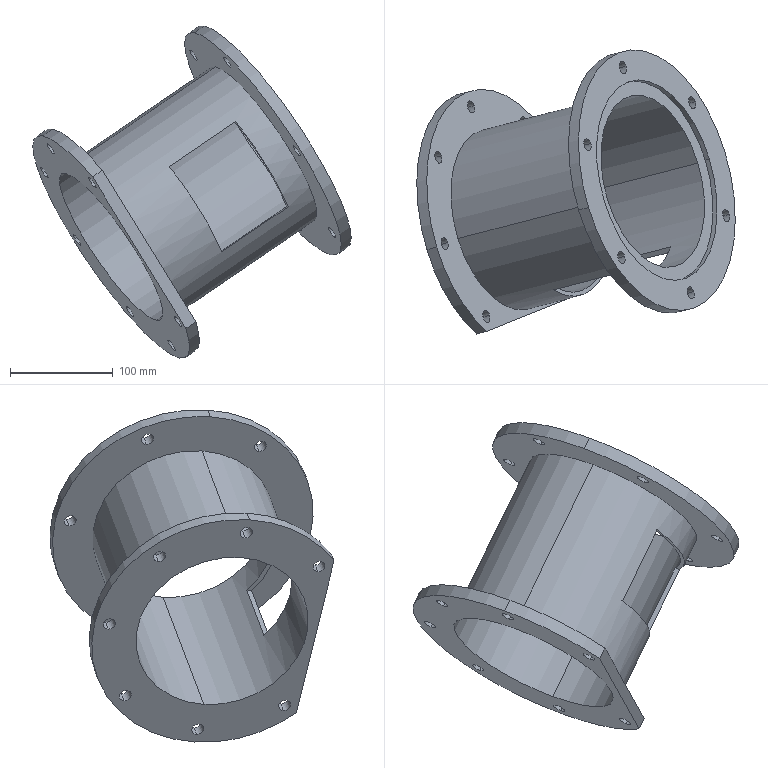Component | SolidWorks | CrusherMotorMount-1 | 1 solid | 47 faces | box 310.61 x 277.08 x 324.38 mm | volume 950992 mm3 | cylinder 37 | plane 10 | commonest cylinder face diameters 12 x26 260 x5 200 x2 180 x2 172 x2
build123d program:
from build123d import *

# Parameters (mm, degrees)
SKETCH2_R          = 6
CUT_EXTRUDE1_DEPTH = 20
CIRPATTERN1_COUNT  = 6
SKETCH3_R          = 100
CUT_EXTRUDE2_DEPTH = 5
CUT_EXTRUDE3_START = -15
SKETCH4_R          = 6
CUT_EXTRUDE3_DEPTH = 15
CIRPATTERN2_COUNT  = 8
SKETCH6_W          = 254.472
SKETCH6_H          = 74.742
CUT_EXTRUDE4_DEPTH = 20
SKETCH7_W          = 80
SKETCH7_H          = 100
CUT_EXTRUDE5_DEPTH = 269.002


with BuildPart() as part:
    # Sketch1 → Revolve1 (revolve)
    with BuildSketch(Plane.XY, mode=Mode.PRIVATE) as revolve1_sk:
        Polygon((0, 86), (0, 130), (12, 130), (12, 90), (183, 90), (183, 130), (195, 130), (195, 86), align=None)
    revolve(revolve1_sk.sketch.rotate(Axis((0, 0, 0), (1, 0, 0)), 90), axis=Axis((0, 0, 0), (1, 0, 0)))

    # Sketch2 → Cut-Extrude1 (cut)
    with BuildSketch(Plane.ZY):
        with Locations((0, 115)):
            Circle(SKETCH2_R)
    cut_extrude1 = extrude(amount=-CUT_EXTRUDE1_DEPTH, mode=Mode.SUBTRACT)

    # CirPattern1: Cut-Extrude1 ×6 about axis
    cirpattern1_axis = Axis((0, 0, 0), (1, 0, 0))
    for i in range(1, CIRPATTERN1_COUNT):
        add(cut_extrude1.rotate(cirpattern1_axis, i * 360 / CIRPATTERN1_COUNT), mode=Mode.SUBTRACT)

    # Sketch3 → Cut-Extrude2 (cut)
    with BuildSketch(Plane.ZY):
        Circle(SKETCH3_R)
    extrude(amount=-CUT_EXTRUDE2_DEPTH, mode=Mode.SUBTRACT)

    # Sketch4 → Cut-Extrude3 (cut)
    with BuildSketch(Plane(origin=(195, 0, 0), x_dir=(0, 0, -1), z_dir=(1, 0, 0)).offset(CUT_EXTRUDE3_START)):
        with Locations(Location((0, 115, 0), (0, 0, 180))):
            Circle(SKETCH4_R)
    cut_extrude3 = extrude(amount=CUT_EXTRUDE3_DEPTH, mode=Mode.SUBTRACT)

    # CirPattern2: Cut-Extrude3 ×8 about axis
    cirpattern2_axis = Axis((0, 0, 0), (1, 0, 0))
    for i in range(1, CIRPATTERN2_COUNT):
        add(cut_extrude3.rotate(cirpattern2_axis, i * 360 / CIRPATTERN2_COUNT), mode=Mode.SUBTRACT)

    # Sketch6 → Cut-Extrude4 (cut)
    with BuildSketch(Plane(origin=(195, 0, 0), x_dir=(0, 0, -1), z_dir=(1, 0, 0))):
        with Locations((20.326, 132.371)):
            Rectangle(SKETCH6_W, SKETCH6_H)
    extrude(amount=-CUT_EXTRUDE4_DEPTH, mode=Mode.SUBTRACT)

    # Sketch7 → Cut-Extrude5 (cut, through all)
    with BuildSketch(Plane(origin=(0, 0, 0), x_dir=(1, 0, 0), z_dir=(0, 1, 0))):
        with Locations((80, 0)):
            Rectangle(SKETCH7_W, SKETCH7_H)
    extrude(amount=CUT_EXTRUDE5_DEPTH, mode=Mode.SUBTRACT)


solid = part.part

# Placed as in the assembly
solid = solid.moved(Location((476.144, -128.045, 108.555), (13.915, -30.844, -160.402)))